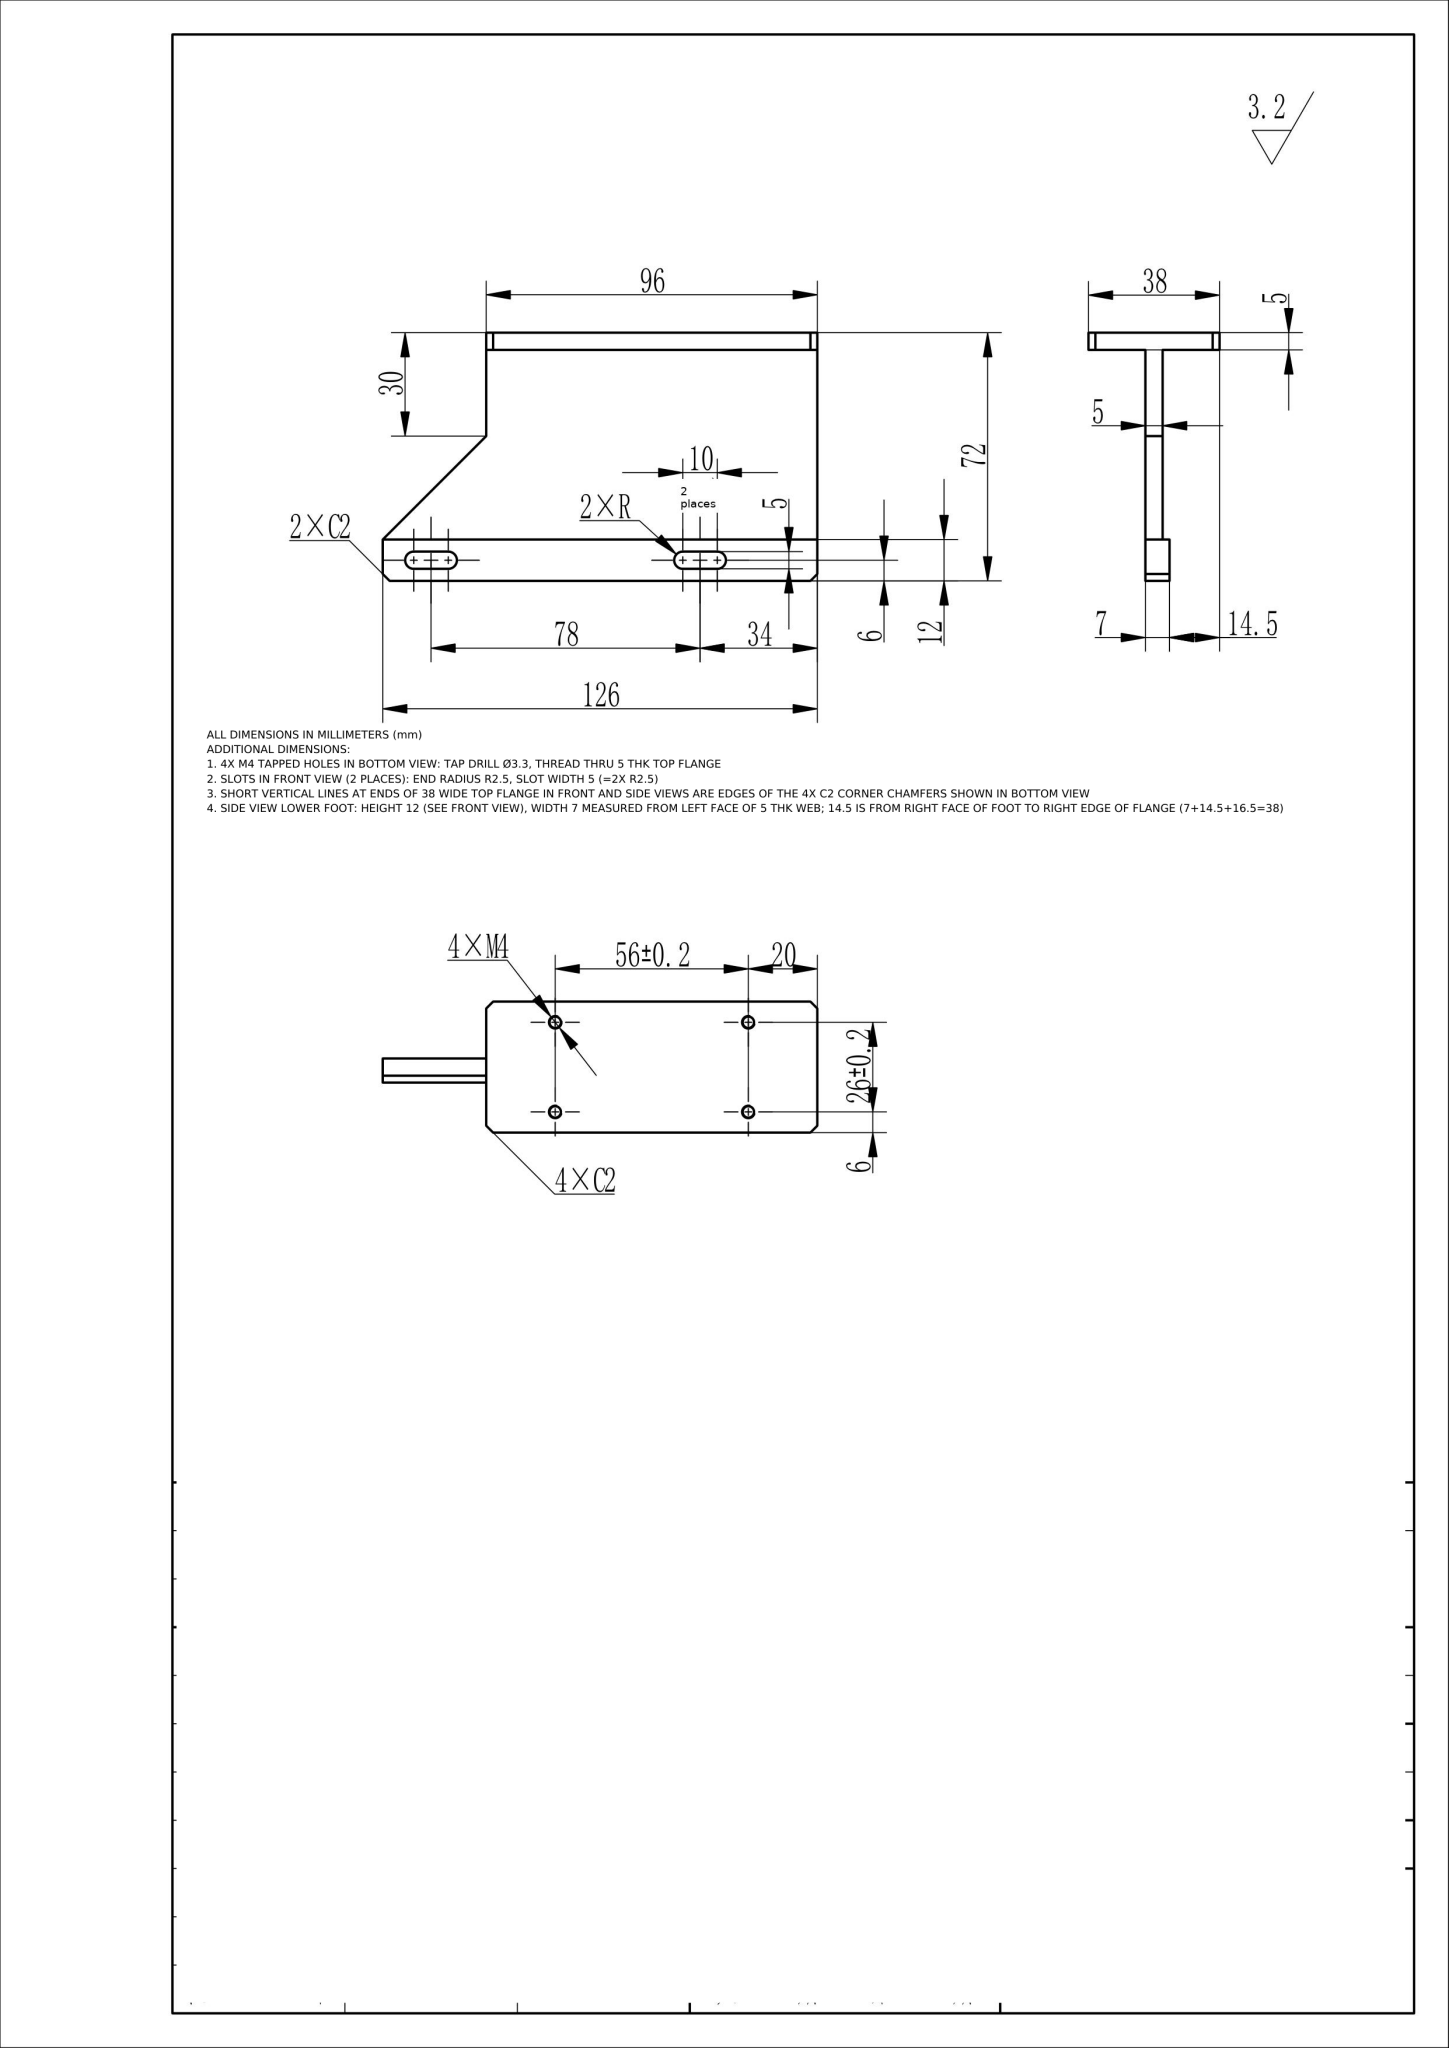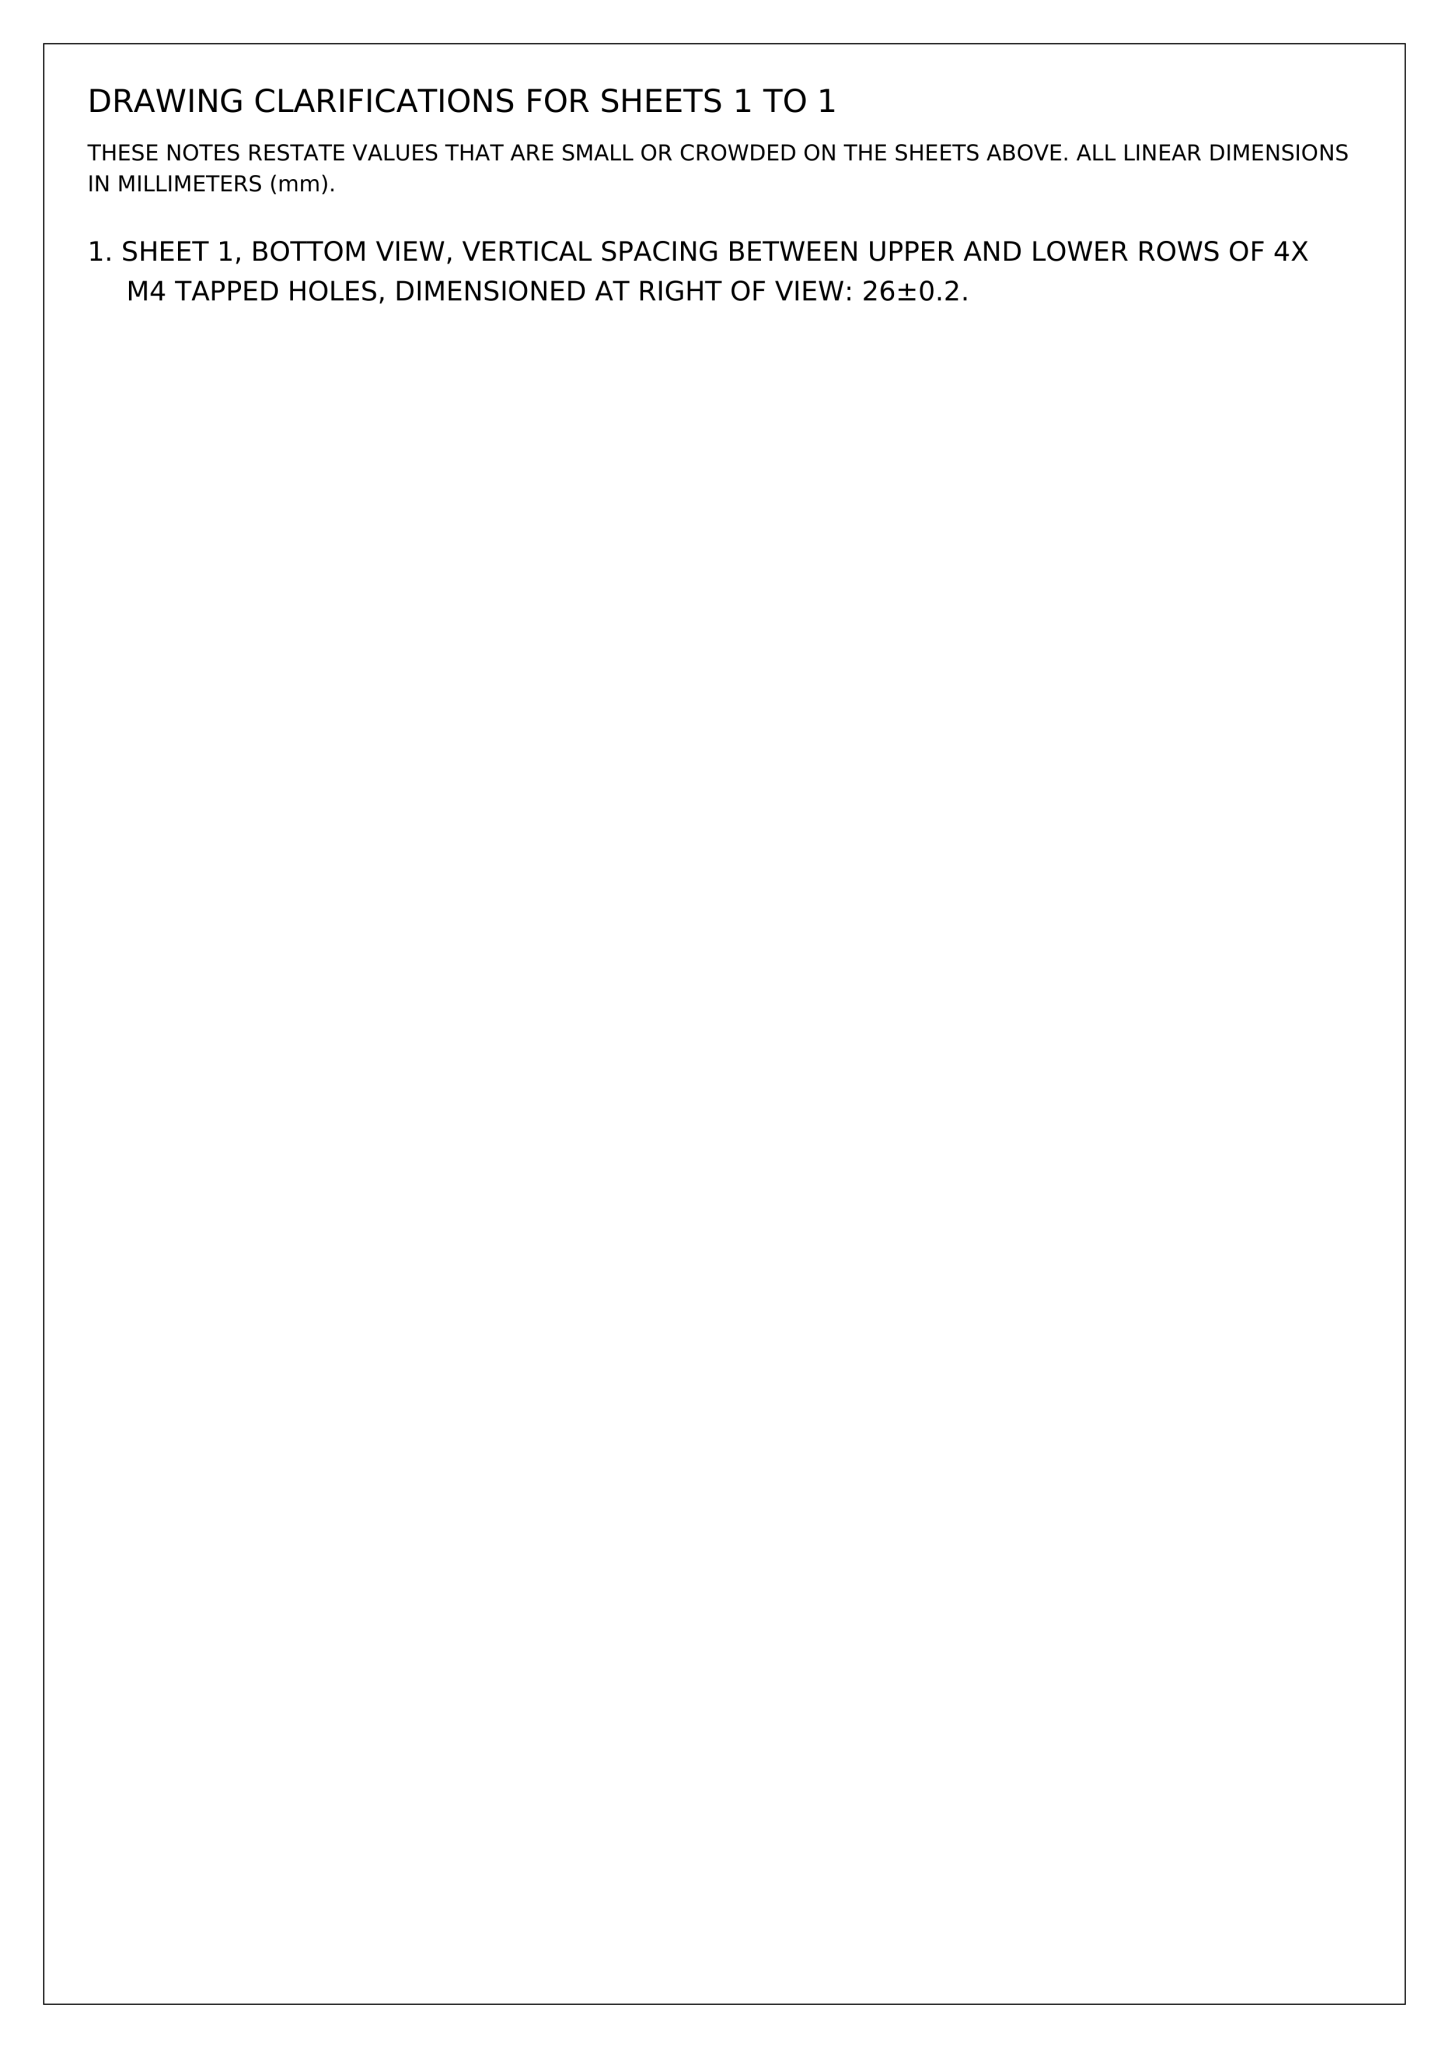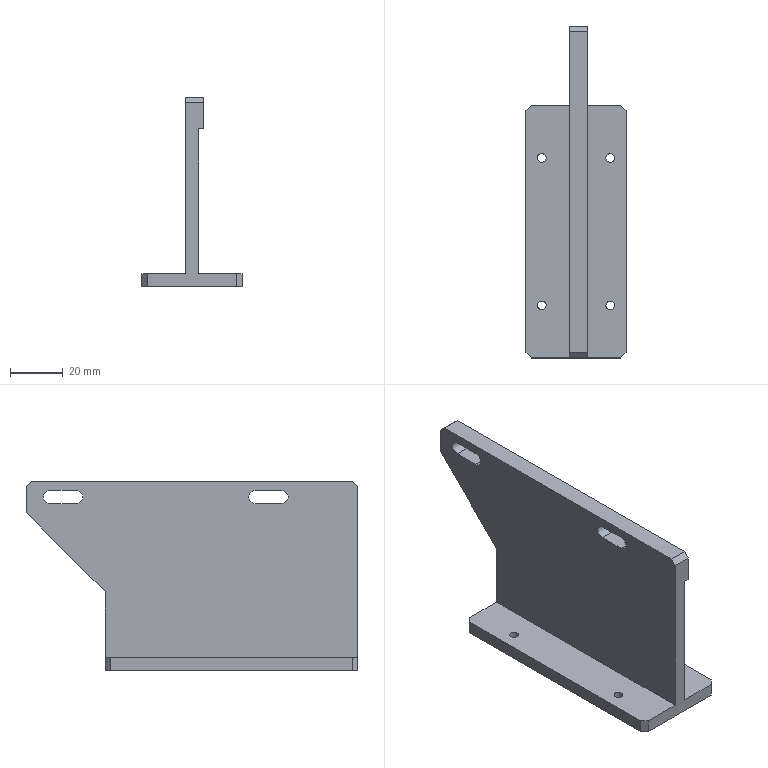Part | NX | mm | 1 solid | 32 faces | box 38 x 126 x 72 mm | volume 56260 mm3 | plane 24 | cylinder 8 | commonest cylinder face diameters 5 x4 3.3 x4